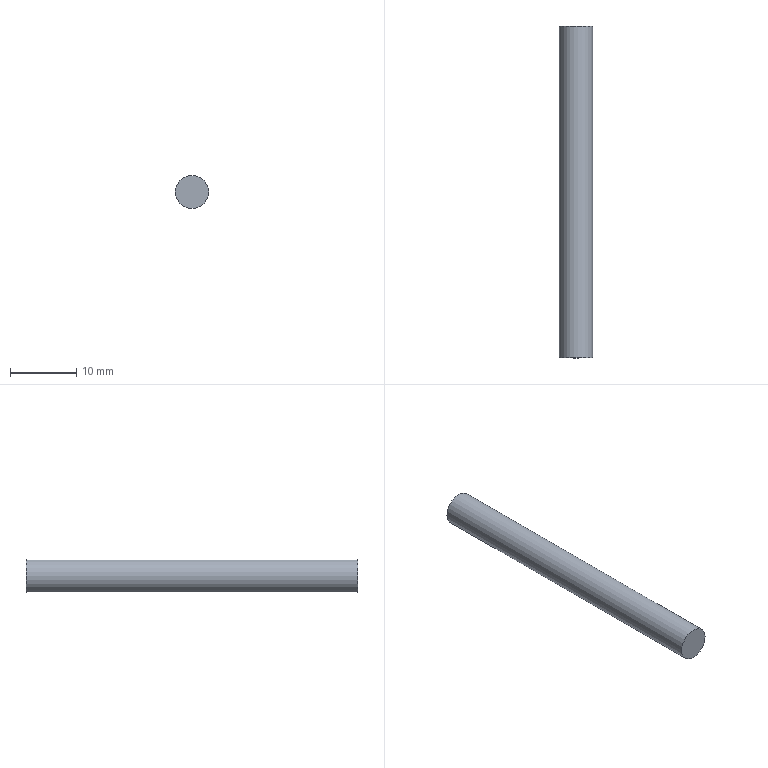Component | NX | CYLINDER_SHAFT | 1 solid | 3 faces | box 5 x 50 x 5 mm | volume 982 mm3 | plane 2 | cylinder 1 | commonest cylinder face diameters 5 x1
STEP:
#1=CARTESIAN_POINT('',(0.,0.,0.));
#2=DIRECTION('',(0.,0.,1.));
#3=DIRECTION('',(1.,0.,0.));
#4=AXIS2_PLACEMENT_3D('',#1,#2,#3);
#5=CARTESIAN_POINT('',(2.5,26.,34.));
#6=VERTEX_POINT('',#5);
#7=CARTESIAN_POINT('',(-0.,26.,34.));
#8=DIRECTION('',(0.,-1.,0.));
#9=DIRECTION('',(1.,0.,0.));
#10=AXIS2_PLACEMENT_3D('',#7,#8,#9);
#11=CIRCLE('',#10,2.5);
#12=CARTESIAN_POINT('',(-0.,26.,34.));
#13=DIRECTION('',(0.,1.,0.));
#14=DIRECTION('',(1.,0.,0.));
#15=AXIS2_PLACEMENT_3D('',#12,#13,#14);
#16=PLANE('',#15);
#17=CARTESIAN_POINT('',(2.5,0.));
#18=CARTESIAN_POINT('',(2.5,-4.33));
#19=CARTESIAN_POINT('',(-1.25,-2.165));
#20=CARTESIAN_POINT('',(-5.,-0.));
#21=CARTESIAN_POINT('',(-1.25,2.165));
#22=CARTESIAN_POINT('',(2.5,4.33));
#23=CARTESIAN_POINT('',(2.5,0.));
#24=(BOUNDED_CURVE()B_SPLINE_CURVE(2,(#17,#18,#19,#20,#21,#22,#23),.UNSPECIFIED.,.T.,.F.)B_SPLINE_CURVE_WITH_KNOTS((1,2,2,2,2,1),(-2.094,0.,2.094,4.189,6.283,8.378),.UNSPECIFIED.)CURVE()GEOMETRIC_REPRESENTATION_ITEM()RATIONAL_B_SPLINE_CURVE((1.,0.5,1.,0.5,1.,0.5,1.))REPRESENTATION_ITEM(''));
#25=(GEOMETRIC_REPRESENTATION_CONTEXT(2)PARAMETRIC_REPRESENTATION_CONTEXT()REPRESENTATION_CONTEXT('',''));
#26=DEFINITIONAL_REPRESENTATION('',(#24),#25);
#27=PCURVE('',#16,#26);
#28=CARTESIAN_POINT('',(-0.,-24.,34.));
#29=DIRECTION('',(0.,1.,0.));
#30=DIRECTION('',(1.,0.,0.));
#31=AXIS2_PLACEMENT_3D('',#28,#29,#30);
#32=CYLINDRICAL_SURFACE('',#31,2.5);
#33=CARTESIAN_POINT('',(6.283,50.));
#34=DIRECTION('',(-1.,0.));
#35=VECTOR('',#34,1.);
#36=LINE('',#33,#35);
#37=(GEOMETRIC_REPRESENTATION_CONTEXT(2)PARAMETRIC_REPRESENTATION_CONTEXT()REPRESENTATION_CONTEXT('',''));
#38=DEFINITIONAL_REPRESENTATION('',(#36),#37);
#39=PCURVE('',#32,#38);
#40=SURFACE_CURVE('',#11,(#27,#39),.PCURVE_S1.);
#41=EDGE_CURVE('',#6,#6,#40,.T.);
#42=ORIENTED_EDGE('',*,*,#41,.F.);
#43=EDGE_LOOP('',(#42));
#44=FACE_BOUND('',#43,.T.);
#45=ADVANCED_FACE('',(#44),#16,.T.);
#46=CARTESIAN_POINT('',(2.5,-24.,34.));
#47=VERTEX_POINT('',#46);
#48=CARTESIAN_POINT('',(-0.,-24.,34.));
#49=DIRECTION('',(0.,1.,0.));
#50=DIRECTION('',(1.,0.,0.));
#51=AXIS2_PLACEMENT_3D('',#48,#49,#50);
#52=CIRCLE('',#51,2.5);
#53=CARTESIAN_POINT('',(-0.,-24.,34.));
#54=DIRECTION('',(0.,-1.,0.));
#55=DIRECTION('',(-1.,0.,0.));
#56=AXIS2_PLACEMENT_3D('',#53,#54,#55);
#57=PLANE('',#56);
#58=CARTESIAN_POINT('',(-2.5,0.));
#59=CARTESIAN_POINT('',(-2.5,4.33));
#60=CARTESIAN_POINT('',(1.25,2.165));
#61=CARTESIAN_POINT('',(5.,0.));
#62=CARTESIAN_POINT('',(1.25,-2.165));
#63=CARTESIAN_POINT('',(-2.5,-4.33));
#64=CARTESIAN_POINT('',(-2.5,0.));
#65=(BOUNDED_CURVE()B_SPLINE_CURVE(2,(#58,#59,#60,#61,#62,#63,#64),.UNSPECIFIED.,.T.,.F.)B_SPLINE_CURVE_WITH_KNOTS((1,2,2,2,2,1),(-2.094,0.,2.094,4.189,6.283,8.378),.UNSPECIFIED.)CURVE()GEOMETRIC_REPRESENTATION_ITEM()RATIONAL_B_SPLINE_CURVE((1.,0.5,1.,0.5,1.,0.5,1.))REPRESENTATION_ITEM(''));
#66=(GEOMETRIC_REPRESENTATION_CONTEXT(2)PARAMETRIC_REPRESENTATION_CONTEXT()REPRESENTATION_CONTEXT('',''));
#67=DEFINITIONAL_REPRESENTATION('',(#65),#66);
#68=PCURVE('',#57,#67);
#69=CARTESIAN_POINT('',(0.,0.));
#70=DIRECTION('',(1.,0.));
#71=VECTOR('',#70,1.);
#72=LINE('',#69,#71);
#73=(GEOMETRIC_REPRESENTATION_CONTEXT(2)PARAMETRIC_REPRESENTATION_CONTEXT()REPRESENTATION_CONTEXT('',''));
#74=DEFINITIONAL_REPRESENTATION('',(#72),#73);
#75=PCURVE('',#32,#74);
#76=SURFACE_CURVE('',#52,(#68,#75),.PCURVE_S1.);
#77=EDGE_CURVE('',#47,#47,#76,.T.);
#78=ORIENTED_EDGE('',*,*,#77,.F.);
#79=EDGE_LOOP('',(#78));
#80=FACE_BOUND('',#79,.T.);
#81=ADVANCED_FACE('',(#80),#57,.T.);
#82=ORIENTED_EDGE('',*,*,#41,.T.);
#83=CARTESIAN_POINT('',(2.5,-24.,34.));
#84=CARTESIAN_POINT('',(2.5,26.,34.));
#85=B_SPLINE_CURVE_WITH_KNOTS('',1,(#83,#84),.UNSPECIFIED.,.F.,.F.,(2,2),(0.,50.),.PIECEWISE_BEZIER_KNOTS.);
#86=CARTESIAN_POINT('',(0.,0.));
#87=DIRECTION('',(0.,1.));
#88=VECTOR('',#87,1.);
#89=LINE('',#86,#88);
#90=(GEOMETRIC_REPRESENTATION_CONTEXT(2)PARAMETRIC_REPRESENTATION_CONTEXT()REPRESENTATION_CONTEXT('',''));
#91=DEFINITIONAL_REPRESENTATION('',(#89),#90);
#92=PCURVE('',#32,#91);
#93=CARTESIAN_POINT('',(6.283,0.));
#94=DIRECTION('',(0.,1.));
#95=VECTOR('',#94,1.);
#96=LINE('',#93,#95);
#97=(GEOMETRIC_REPRESENTATION_CONTEXT(2)PARAMETRIC_REPRESENTATION_CONTEXT()REPRESENTATION_CONTEXT('',''));
#98=DEFINITIONAL_REPRESENTATION('',(#96),#97);
#99=PCURVE('',#32,#98);
#100=SEAM_CURVE('',#85,(#92,#99),.PCURVE_S1.);
#101=EDGE_CURVE('',#47,#6,#100,.T.);
#102=ORIENTED_EDGE('',*,*,#101,.F.);
#103=ORIENTED_EDGE('',*,*,#77,.T.);
#104=ORIENTED_EDGE('',*,*,#101,.T.);
#105=EDGE_LOOP('',(#82,#102,#103,#104));
#106=FACE_BOUND('',#105,.T.);
#107=ADVANCED_FACE('',(#106),#32,.T.);
#108=CLOSED_SHELL('',(#45,#81,#107));
#109=MANIFOLD_SOLID_BREP('',#108);
#110=(LENGTH_UNIT()NAMED_UNIT(*)SI_UNIT(.MILLI.,.METRE.));
#111=UNCERTAINTY_MEASURE_WITH_UNIT(LENGTH_MEASURE(0.00001),#110,'','');
#112=(NAMED_UNIT(*)PLANE_ANGLE_UNIT()SI_UNIT($,.RADIAN.));
#113=(NAMED_UNIT(*)SI_UNIT($,.STERADIAN.)SOLID_ANGLE_UNIT());
#114=(GEOMETRIC_REPRESENTATION_CONTEXT(3)GLOBAL_UNCERTAINTY_ASSIGNED_CONTEXT((#111))GLOBAL_UNIT_ASSIGNED_CONTEXT((#110,#112,#113))REPRESENTATION_CONTEXT('',''));
#115=ADVANCED_BREP_SHAPE_REPRESENTATION('',(#4,#109),#114);